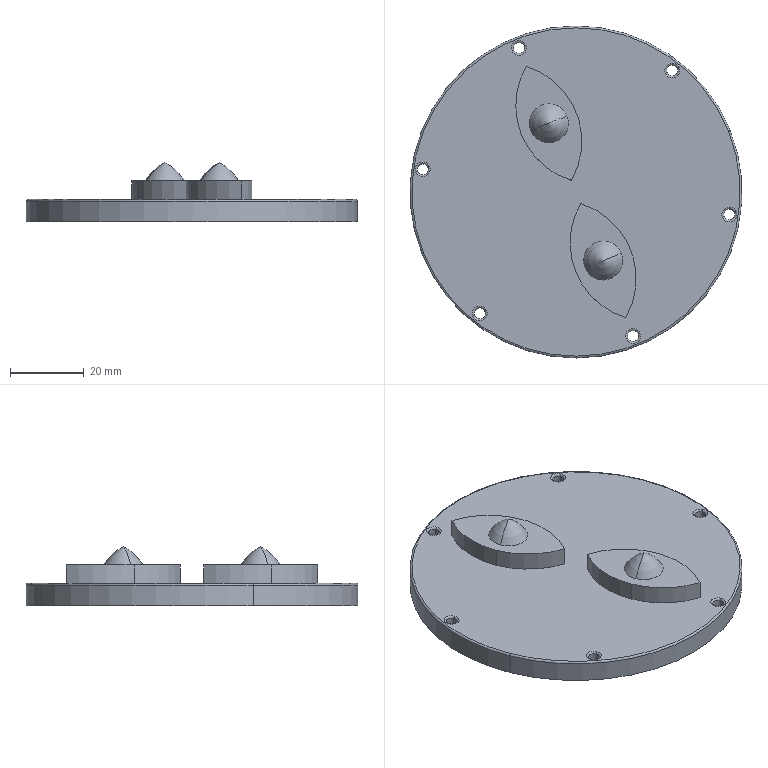Component | SolidWorks | JawCover-1 | 1 solid | 42 faces | volume 41999 mm3 | cylinder 20 | torus 18 | plane 4 | commonest cylinder face diameters 3 x12 42.46 x6 90 x2